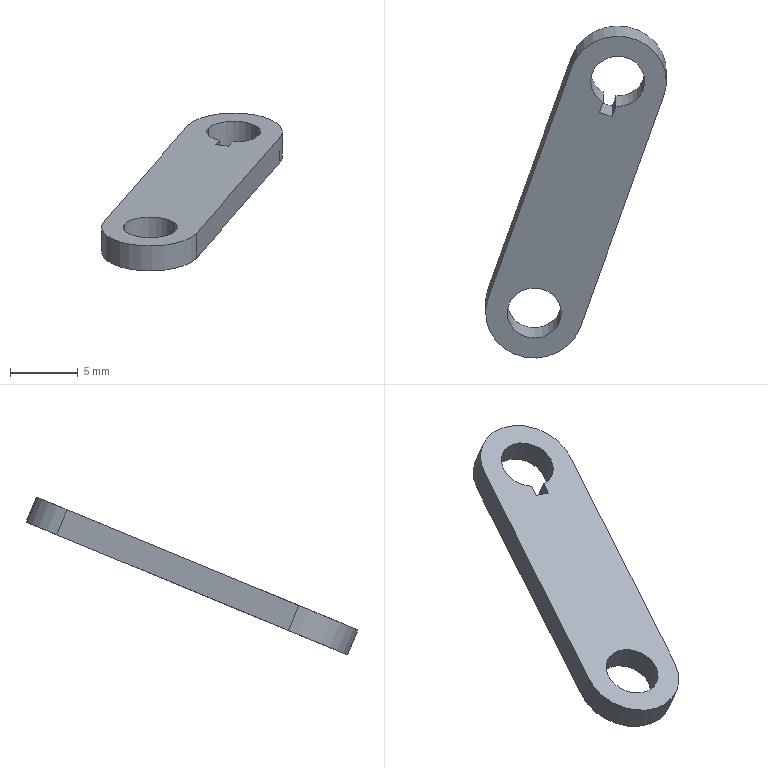Component | SolidWorks | MirrorShort Arm-2 | 1 solid | 14 faces | box 13.38 x 24.55 x 11.68 mm | volume 311 mm3 | cylinder 7 | plane 7 | commonest cylinder face diameters 4 x5 7.2 x2
STEP:
#1=CARTESIAN_POINT('',(12.305,-1.564,2.111));
#2=VERTEX_POINT('',#1);
#3=CARTESIAN_POINT('',(12.454,-1.61,2.092));
#4=VERTEX_POINT('',#3);
#5=CARTESIAN_POINT('',(12.38,-1.587,2.101));
#6=DIRECTION('',(-0.,-0.3818,0.9242));
#7=DIRECTION('',(-0.9487,0.2921,0.1207));
#8=AXIS2_PLACEMENT_3D('',#5,#6,#7);
#9=CIRCLE('',#8,0.07874);
#10=EDGE_CURVE('',#2,#4,#9,.T.);
#11=ORIENTED_EDGE('',*,*,#10,.F.);
#12=CARTESIAN_POINT('',(12.305,-1.594,2.183));
#13=VERTEX_POINT('',#12);
#14=CARTESIAN_POINT('',(12.305,-1.564,2.111));
#15=DIRECTION('',(-0.,-0.3818,0.9242));
#16=VECTOR('',#15,39.37);
#17=LINE('',#14,#16);
#18=EDGE_CURVE('',#2,#13,#17,.T.);
#19=ORIENTED_EDGE('',*,*,#18,.T.);
#20=CARTESIAN_POINT('',(12.454,-1.64,2.164));
#21=VERTEX_POINT('',#20);
#22=CARTESIAN_POINT('',(12.38,-1.617,2.174));
#23=DIRECTION('',(-0.,-0.3818,0.9242));
#24=DIRECTION('',(-0.9487,0.2921,0.1207));
#25=AXIS2_PLACEMENT_3D('',#22,#23,#24);
#26=CIRCLE('',#25,0.07874);
#27=EDGE_CURVE('',#13,#21,#26,.T.);
#28=ORIENTED_EDGE('',*,*,#27,.T.);
#29=CARTESIAN_POINT('',(12.454,-1.61,2.092));
#30=DIRECTION('',(-0.,-0.3818,0.9242));
#31=VECTOR('',#30,39.37);
#32=LINE('',#29,#31);
#33=EDGE_CURVE('',#4,#21,#32,.T.);
#34=ORIENTED_EDGE('',*,*,#33,.F.);
#35=EDGE_LOOP('',(#11,#19,#28,#34));
#36=FACE_OUTER_BOUND('',#35,.T.);
#37=CARTESIAN_POINT('',(12.38,-1.587,2.101));
#38=DIRECTION('',(-0.,-0.3818,0.9242));
#39=DIRECTION('',(0.9487,-0.2921,-0.1207));
#40=AXIS2_PLACEMENT_3D('',#37,#38,#39);
#41=CYLINDRICAL_SURFACE('',#40,0.07874);
#42=ADVANCED_FACE('',(#36),#41,.F.);
#43=CARTESIAN_POINT('',(12.548,-0.8897,2.389));
#44=VERTEX_POINT('',#43);
#45=CARTESIAN_POINT('',(12.58,-0.9738,2.354));
#46=VERTEX_POINT('',#45);
#47=CARTESIAN_POINT('',(12.623,-0.9127,2.38));
#48=DIRECTION('',(-0.,-0.3818,0.9242));
#49=DIRECTION('',(-0.9487,0.2921,0.1207));
#50=AXIS2_PLACEMENT_3D('',#47,#48,#49);
#51=CIRCLE('',#50,0.07874);
#52=EDGE_CURVE('',#44,#46,#51,.T.);
#53=ORIENTED_EDGE('',*,*,#52,.F.);
#54=CARTESIAN_POINT('',(12.548,-0.9197,2.462));
#55=VERTEX_POINT('',#54);
#56=CARTESIAN_POINT('',(12.548,-0.8897,2.389));
#57=DIRECTION('',(-0.,-0.3818,0.9242));
#58=VECTOR('',#57,39.37);
#59=LINE('',#56,#58);
#60=EDGE_CURVE('',#44,#55,#59,.T.);
#61=ORIENTED_EDGE('',*,*,#60,.T.);
#62=CARTESIAN_POINT('',(12.58,-1.004,2.427));
#63=VERTEX_POINT('',#62);
#64=CARTESIAN_POINT('',(12.623,-0.9427,2.452));
#65=DIRECTION('',(-0.,-0.3818,0.9242));
#66=DIRECTION('',(-0.9487,0.2921,0.1207));
#67=AXIS2_PLACEMENT_3D('',#64,#65,#66);
#68=CIRCLE('',#67,0.07874);
#69=EDGE_CURVE('',#55,#63,#68,.T.);
#70=ORIENTED_EDGE('',*,*,#69,.T.);
#71=CARTESIAN_POINT('',(12.58,-0.9738,2.354));
#72=DIRECTION('',(0.,0.3818,-0.9242));
#73=VECTOR('',#72,39.37);
#74=LINE('',#71,#73);
#75=EDGE_CURVE('',#63,#46,#74,.T.);
#76=ORIENTED_EDGE('',*,*,#75,.T.);
#77=EDGE_LOOP('',(#53,#61,#70,#76));
#78=FACE_OUTER_BOUND('',#77,.T.);
#79=CARTESIAN_POINT('',(12.623,-0.9127,2.38));
#80=DIRECTION('',(-0.,-0.3818,0.9242));
#81=DIRECTION('',(0.9487,-0.2921,-0.1207));
#82=AXIS2_PLACEMENT_3D('',#79,#80,#81);
#83=CYLINDRICAL_SURFACE('',#82,0.07874);
#84=ADVANCED_FACE('',(#78),#83,.F.);
#85=ORIENTED_EDGE('',*,*,#60,.F.);
#86=CARTESIAN_POINT('',(12.698,-0.9357,2.37));
#87=VERTEX_POINT('',#86);
#88=CARTESIAN_POINT('',(12.623,-0.9127,2.38));
#89=DIRECTION('',(-0.,-0.3818,0.9242));
#90=DIRECTION('',(-0.9487,0.2921,0.1207));
#91=AXIS2_PLACEMENT_3D('',#88,#89,#90);
#92=CIRCLE('',#91,0.07874);
#93=EDGE_CURVE('',#87,#44,#92,.T.);
#94=ORIENTED_EDGE('',*,*,#93,.F.);
#95=CARTESIAN_POINT('',(12.698,-0.9657,2.443));
#96=VERTEX_POINT('',#95);
#97=CARTESIAN_POINT('',(12.698,-0.9357,2.37));
#98=DIRECTION('',(-0.,-0.3818,0.9242));
#99=VECTOR('',#98,39.37);
#100=LINE('',#97,#99);
#101=EDGE_CURVE('',#87,#96,#100,.T.);
#102=ORIENTED_EDGE('',*,*,#101,.T.);
#103=CARTESIAN_POINT('',(12.623,-0.9427,2.452));
#104=DIRECTION('',(-0.,-0.3818,0.9242));
#105=DIRECTION('',(-0.9487,0.2921,0.1207));
#106=AXIS2_PLACEMENT_3D('',#103,#104,#105);
#107=CIRCLE('',#106,0.07874);
#108=EDGE_CURVE('',#96,#55,#107,.T.);
#109=ORIENTED_EDGE('',*,*,#108,.T.);
#110=EDGE_LOOP('',(#85,#94,#102,#109));
#111=FACE_OUTER_BOUND('',#110,.T.);
#112=CARTESIAN_POINT('',(12.623,-0.9127,2.38));
#113=DIRECTION('',(-0.,-0.3818,0.9242));
#114=DIRECTION('',(0.9487,-0.2921,-0.1207));
#115=AXIS2_PLACEMENT_3D('',#112,#113,#114);
#116=CYLINDRICAL_SURFACE('',#115,0.07874);
#117=ADVANCED_FACE('',(#111),#116,.F.);
#118=CARTESIAN_POINT('',(12.607,-1.015,2.337));
#119=VERTEX_POINT('',#118);
#120=CARTESIAN_POINT('',(12.617,-0.9853,2.35));
#121=VERTEX_POINT('',#120);
#122=CARTESIAN_POINT('',(12.642,-0.9184,2.377));
#123=DIRECTION('',(0.3161,0.8768,0.3623));
#124=VECTOR('',#123,39.37);
#125=LINE('',#122,#124);
#126=EDGE_CURVE('',#119,#121,#125,.T.);
#127=ORIENTED_EDGE('',*,*,#126,.T.);
#128=CARTESIAN_POINT('',(12.623,-0.9127,2.38));
#129=DIRECTION('',(-0.,-0.3818,0.9242));
#130=DIRECTION('',(-0.9487,0.2921,0.1207));
#131=AXIS2_PLACEMENT_3D('',#128,#129,#130);
#132=CIRCLE('',#131,0.07874);
#133=EDGE_CURVE('',#121,#87,#132,.T.);
#134=ORIENTED_EDGE('',*,*,#133,.T.);
#135=ORIENTED_EDGE('',*,*,#93,.T.);
#136=ORIENTED_EDGE('',*,*,#52,.T.);
#137=CARTESIAN_POINT('',(12.569,-1.004,2.342));
#138=VERTEX_POINT('',#137);
#139=CARTESIAN_POINT('',(12.604,-0.9069,2.382));
#140=DIRECTION('',(-0.3161,-0.8768,-0.3623));
#141=VECTOR('',#140,39.37);
#142=LINE('',#139,#141);
#143=EDGE_CURVE('',#46,#138,#142,.T.);
#144=ORIENTED_EDGE('',*,*,#143,.T.);
#145=CARTESIAN_POINT('',(12.588,-1.009,2.34));
#146=DIRECTION('',(0.9487,-0.2921,-0.1207));
#147=VECTOR('',#146,39.37);
#148=LINE('',#145,#147);
#149=EDGE_CURVE('',#138,#119,#148,.T.);
#150=ORIENTED_EDGE('',*,*,#149,.T.);
#151=EDGE_LOOP('',(#127,#134,#135,#136,#144,#150));
#152=FACE_BOUND('',#151,.T.);
#153=CARTESIAN_POINT('',(12.757,-0.9541,2.363));
#154=VERTEX_POINT('',#153);
#155=CARTESIAN_POINT('',(12.488,-0.8713,2.397));
#156=VERTEX_POINT('',#155);
#157=CARTESIAN_POINT('',(12.623,-0.9127,2.38));
#158=DIRECTION('',(-0.,-0.3818,0.9242));
#159=DIRECTION('',(-0.9487,0.2921,0.1207));
#160=AXIS2_PLACEMENT_3D('',#157,#158,#159);
#161=CIRCLE('',#160,0.1417);
#162=EDGE_CURVE('',#154,#156,#161,.T.);
#163=ORIENTED_EDGE('',*,*,#162,.F.);
#164=CARTESIAN_POINT('',(12.514,-1.629,2.084));
#165=VERTEX_POINT('',#164);
#166=CARTESIAN_POINT('',(12.757,-0.9541,2.363));
#167=DIRECTION('',(0.3161,0.8768,0.3623));
#168=VECTOR('',#167,39.37);
#169=LINE('',#166,#168);
#170=EDGE_CURVE('',#165,#154,#169,.T.);
#171=ORIENTED_EDGE('',*,*,#170,.F.);
#172=CARTESIAN_POINT('',(12.245,-1.546,2.118));
#173=VERTEX_POINT('',#172);
#174=CARTESIAN_POINT('',(12.38,-1.587,2.101));
#175=DIRECTION('',(-0.,-0.3818,0.9242));
#176=DIRECTION('',(-0.9487,0.2921,0.1207));
#177=AXIS2_PLACEMENT_3D('',#174,#175,#176);
#178=CIRCLE('',#177,0.1417);
#179=EDGE_CURVE('',#173,#165,#178,.T.);
#180=ORIENTED_EDGE('',*,*,#179,.F.);
#181=CARTESIAN_POINT('',(12.488,-0.8713,2.397));
#182=DIRECTION('',(-0.3161,-0.8768,-0.3623));
#183=VECTOR('',#182,39.37);
#184=LINE('',#181,#183);
#185=EDGE_CURVE('',#156,#173,#184,.T.);
#186=ORIENTED_EDGE('',*,*,#185,.F.);
#187=EDGE_LOOP('',(#163,#171,#180,#186));
#188=FACE_OUTER_BOUND('',#187,.T.);
#189=CARTESIAN_POINT('',(12.38,-1.587,2.101));
#190=DIRECTION('',(-0.,-0.3818,0.9242));
#191=DIRECTION('',(-0.9487,0.2921,0.1207));
#192=AXIS2_PLACEMENT_3D('',#189,#190,#191);
#193=CIRCLE('',#192,0.07874);
#194=EDGE_CURVE('',#4,#2,#193,.T.);
#195=ORIENTED_EDGE('',*,*,#194,.T.);
#196=ORIENTED_EDGE('',*,*,#10,.T.);
#197=EDGE_LOOP('',(#195,#196));
#198=FACE_BOUND('',#197,.T.);
#199=CARTESIAN_POINT('',(12.623,-0.9127,2.38));
#200=DIRECTION('',(0.,0.3818,-0.9242));
#201=DIRECTION('',(-0.9487,0.2921,0.1207));
#202=AXIS2_PLACEMENT_3D('',#199,#200,#201);
#203=PLANE('',#202);
#204=ADVANCED_FACE('',(#152,#188,#198),#203,.T.);
#205=CARTESIAN_POINT('',(12.757,-0.9841,2.435));
#206=VERTEX_POINT('',#205);
#207=CARTESIAN_POINT('',(12.488,-0.9013,2.47));
#208=VERTEX_POINT('',#207);
#209=CARTESIAN_POINT('',(12.623,-0.9427,2.452));
#210=DIRECTION('',(-0.,-0.3818,0.9242));
#211=DIRECTION('',(-0.9487,0.2921,0.1207));
#212=AXIS2_PLACEMENT_3D('',#209,#210,#211);
#213=CIRCLE('',#212,0.1417);
#214=EDGE_CURVE('',#206,#208,#213,.T.);
#215=ORIENTED_EDGE('',*,*,#214,.T.);
#216=CARTESIAN_POINT('',(12.245,-1.576,2.191));
#217=VERTEX_POINT('',#216);
#218=CARTESIAN_POINT('',(12.488,-0.9013,2.47));
#219=DIRECTION('',(-0.3161,-0.8768,-0.3623));
#220=VECTOR('',#219,39.37);
#221=LINE('',#218,#220);
#222=EDGE_CURVE('',#208,#217,#221,.T.);
#223=ORIENTED_EDGE('',*,*,#222,.T.);
#224=CARTESIAN_POINT('',(12.514,-1.659,2.157));
#225=VERTEX_POINT('',#224);
#226=CARTESIAN_POINT('',(12.38,-1.617,2.174));
#227=DIRECTION('',(-0.,-0.3818,0.9242));
#228=DIRECTION('',(-0.9487,0.2921,0.1207));
#229=AXIS2_PLACEMENT_3D('',#226,#227,#228);
#230=CIRCLE('',#229,0.1417);
#231=EDGE_CURVE('',#217,#225,#230,.T.);
#232=ORIENTED_EDGE('',*,*,#231,.T.);
#233=CARTESIAN_POINT('',(12.757,-0.9841,2.435));
#234=DIRECTION('',(0.3161,0.8768,0.3623));
#235=VECTOR('',#234,39.37);
#236=LINE('',#233,#235);
#237=EDGE_CURVE('',#225,#206,#236,.T.);
#238=ORIENTED_EDGE('',*,*,#237,.T.);
#239=EDGE_LOOP('',(#215,#223,#232,#238));
#240=FACE_OUTER_BOUND('',#239,.T.);
#241=CARTESIAN_POINT('',(12.569,-1.034,2.415));
#242=VERTEX_POINT('',#241);
#243=CARTESIAN_POINT('',(12.607,-1.045,2.41));
#244=VERTEX_POINT('',#243);
#245=CARTESIAN_POINT('',(12.607,-1.045,2.41));
#246=DIRECTION('',(0.9487,-0.2921,-0.1207));
#247=VECTOR('',#246,39.37);
#248=LINE('',#245,#247);
#249=EDGE_CURVE('',#242,#244,#248,.T.);
#250=ORIENTED_EDGE('',*,*,#249,.F.);
#251=CARTESIAN_POINT('',(12.604,-0.937,2.455));
#252=DIRECTION('',(-0.3161,-0.8768,-0.3623));
#253=VECTOR('',#252,39.37);
#254=LINE('',#251,#253);
#255=EDGE_CURVE('',#63,#242,#254,.T.);
#256=ORIENTED_EDGE('',*,*,#255,.F.);
#257=ORIENTED_EDGE('',*,*,#69,.F.);
#258=ORIENTED_EDGE('',*,*,#108,.F.);
#259=CARTESIAN_POINT('',(12.617,-1.015,2.422));
#260=VERTEX_POINT('',#259);
#261=CARTESIAN_POINT('',(12.623,-0.9427,2.452));
#262=DIRECTION('',(-0.,-0.3818,0.9242));
#263=DIRECTION('',(-0.9487,0.2921,0.1207));
#264=AXIS2_PLACEMENT_3D('',#261,#262,#263);
#265=CIRCLE('',#264,0.07874);
#266=EDGE_CURVE('',#260,#96,#265,.T.);
#267=ORIENTED_EDGE('',*,*,#266,.F.);
#268=CARTESIAN_POINT('',(12.642,-0.9485,2.45));
#269=DIRECTION('',(0.3161,0.8768,0.3623));
#270=VECTOR('',#269,39.37);
#271=LINE('',#268,#270);
#272=EDGE_CURVE('',#244,#260,#271,.T.);
#273=ORIENTED_EDGE('',*,*,#272,.F.);
#274=EDGE_LOOP('',(#250,#256,#257,#258,#267,#273));
#275=FACE_BOUND('',#274,.T.);
#276=CARTESIAN_POINT('',(12.38,-1.617,2.174));
#277=DIRECTION('',(-0.,-0.3818,0.9242));
#278=DIRECTION('',(-0.9487,0.2921,0.1207));
#279=AXIS2_PLACEMENT_3D('',#276,#277,#278);
#280=CIRCLE('',#279,0.07874);
#281=EDGE_CURVE('',#21,#13,#280,.T.);
#282=ORIENTED_EDGE('',*,*,#281,.F.);
#283=ORIENTED_EDGE('',*,*,#27,.F.);
#284=EDGE_LOOP('',(#282,#283));
#285=FACE_BOUND('',#284,.T.);
#286=CARTESIAN_POINT('',(12.623,-0.9427,2.452));
#287=DIRECTION('',(0.,0.3818,-0.9242));
#288=DIRECTION('',(-0.9487,0.2921,0.1207));
#289=AXIS2_PLACEMENT_3D('',#286,#287,#288);
#290=PLANE('',#289);
#291=ADVANCED_FACE('',(#240,#275,#285),#290,.F.);
#292=ORIENTED_EDGE('',*,*,#214,.F.);
#293=CARTESIAN_POINT('',(12.757,-0.9541,2.363));
#294=DIRECTION('',(-0.,-0.3818,0.9242));
#295=VECTOR('',#294,39.37);
#296=LINE('',#293,#295);
#297=EDGE_CURVE('',#154,#206,#296,.T.);
#298=ORIENTED_EDGE('',*,*,#297,.F.);
#299=ORIENTED_EDGE('',*,*,#162,.T.);
#300=CARTESIAN_POINT('',(12.488,-0.8713,2.397));
#301=DIRECTION('',(-0.,-0.3818,0.9242));
#302=VECTOR('',#301,39.37);
#303=LINE('',#300,#302);
#304=EDGE_CURVE('',#156,#208,#303,.T.);
#305=ORIENTED_EDGE('',*,*,#304,.T.);
#306=EDGE_LOOP('',(#292,#298,#299,#305));
#307=FACE_OUTER_BOUND('',#306,.T.);
#308=CARTESIAN_POINT('',(12.623,-0.9127,2.38));
#309=DIRECTION('',(-0.,-0.3818,0.9242));
#310=DIRECTION('',(0.9487,-0.2921,-0.1207));
#311=AXIS2_PLACEMENT_3D('',#308,#309,#310);
#312=CYLINDRICAL_SURFACE('',#311,0.1417);
#313=ADVANCED_FACE('',(#307),#312,.T.);
#314=ORIENTED_EDGE('',*,*,#222,.F.);
#315=ORIENTED_EDGE('',*,*,#304,.F.);
#316=ORIENTED_EDGE('',*,*,#185,.T.);
#317=CARTESIAN_POINT('',(12.245,-1.546,2.118));
#318=DIRECTION('',(-0.,-0.3818,0.9242));
#319=VECTOR('',#318,39.37);
#320=LINE('',#317,#319);
#321=EDGE_CURVE('',#173,#217,#320,.T.);
#322=ORIENTED_EDGE('',*,*,#321,.T.);
#323=EDGE_LOOP('',(#314,#315,#316,#322));
#324=FACE_OUTER_BOUND('',#323,.T.);
#325=CARTESIAN_POINT('',(12.488,-0.8713,2.397));
#326=DIRECTION('',(0.9487,-0.2921,-0.1207));
#327=DIRECTION('',(0.3161,0.8768,0.3623));
#328=AXIS2_PLACEMENT_3D('',#325,#326,#327);
#329=PLANE('',#328);
#330=ADVANCED_FACE('',(#324),#329,.F.);
#331=ORIENTED_EDGE('',*,*,#231,.F.);
#332=ORIENTED_EDGE('',*,*,#321,.F.);
#333=ORIENTED_EDGE('',*,*,#179,.T.);
#334=CARTESIAN_POINT('',(12.514,-1.629,2.084));
#335=DIRECTION('',(-0.,-0.3818,0.9242));
#336=VECTOR('',#335,39.37);
#337=LINE('',#334,#336);
#338=EDGE_CURVE('',#165,#225,#337,.T.);
#339=ORIENTED_EDGE('',*,*,#338,.T.);
#340=EDGE_LOOP('',(#331,#332,#333,#339));
#341=FACE_OUTER_BOUND('',#340,.T.);
#342=CARTESIAN_POINT('',(12.38,-1.587,2.101));
#343=DIRECTION('',(-0.,-0.3818,0.9242));
#344=DIRECTION('',(0.9487,-0.2921,-0.1207));
#345=AXIS2_PLACEMENT_3D('',#342,#343,#344);
#346=CYLINDRICAL_SURFACE('',#345,0.1417);
#347=ADVANCED_FACE('',(#341),#346,.T.);
#348=ORIENTED_EDGE('',*,*,#237,.F.);
#349=ORIENTED_EDGE('',*,*,#338,.F.);
#350=ORIENTED_EDGE('',*,*,#170,.T.);
#351=ORIENTED_EDGE('',*,*,#297,.T.);
#352=EDGE_LOOP('',(#348,#349,#350,#351));
#353=FACE_OUTER_BOUND('',#352,.T.);
#354=CARTESIAN_POINT('',(12.757,-0.9541,2.363));
#355=DIRECTION('',(-0.9487,0.2921,0.1207));
#356=DIRECTION('',(-0.3161,-0.8768,-0.3623));
#357=AXIS2_PLACEMENT_3D('',#354,#355,#356);
#358=PLANE('',#357);
#359=ADVANCED_FACE('',(#353),#358,.F.);
#360=ORIENTED_EDGE('',*,*,#101,.F.);
#361=ORIENTED_EDGE('',*,*,#133,.F.);
#362=CARTESIAN_POINT('',(12.617,-0.9853,2.35));
#363=DIRECTION('',(-0.,-0.3818,0.9242));
#364=VECTOR('',#363,39.37);
#365=LINE('',#362,#364);
#366=EDGE_CURVE('',#121,#260,#365,.T.);
#367=ORIENTED_EDGE('',*,*,#366,.T.);
#368=ORIENTED_EDGE('',*,*,#266,.T.);
#369=EDGE_LOOP('',(#360,#361,#367,#368));
#370=FACE_OUTER_BOUND('',#369,.T.);
#371=CARTESIAN_POINT('',(12.623,-0.9127,2.38));
#372=DIRECTION('',(-0.,-0.3818,0.9242));
#373=DIRECTION('',(0.9487,-0.2921,-0.1207));
#374=AXIS2_PLACEMENT_3D('',#371,#372,#373);
#375=CYLINDRICAL_SURFACE('',#374,0.07874);
#376=ADVANCED_FACE('',(#370),#375,.F.);
#377=ORIENTED_EDGE('',*,*,#18,.F.);
#378=ORIENTED_EDGE('',*,*,#194,.F.);
#379=ORIENTED_EDGE('',*,*,#33,.T.);
#380=ORIENTED_EDGE('',*,*,#281,.T.);
#381=EDGE_LOOP('',(#377,#378,#379,#380));
#382=FACE_OUTER_BOUND('',#381,.T.);
#383=CARTESIAN_POINT('',(12.38,-1.587,2.101));
#384=DIRECTION('',(-0.,-0.3818,0.9242));
#385=DIRECTION('',(0.9487,-0.2921,-0.1207));
#386=AXIS2_PLACEMENT_3D('',#383,#384,#385);
#387=CYLINDRICAL_SURFACE('',#386,0.07874);
#388=ADVANCED_FACE('',(#382),#387,.F.);
#389=ORIENTED_EDGE('',*,*,#126,.F.);
#390=CARTESIAN_POINT('',(12.607,-1.045,2.41));
#391=DIRECTION('',(0.,0.3818,-0.9242));
#392=VECTOR('',#391,39.37);
#393=LINE('',#390,#392);
#394=EDGE_CURVE('',#244,#119,#393,.T.);
#395=ORIENTED_EDGE('',*,*,#394,.F.);
#396=ORIENTED_EDGE('',*,*,#272,.T.);
#397=ORIENTED_EDGE('',*,*,#366,.F.);
#398=EDGE_LOOP('',(#389,#395,#396,#397));
#399=FACE_OUTER_BOUND('',#398,.T.);
#400=CARTESIAN_POINT('',(12.642,-0.9485,2.45));
#401=DIRECTION('',(0.9487,-0.2921,-0.1207));
#402=DIRECTION('',(0.3161,0.8768,0.3623));
#403=AXIS2_PLACEMENT_3D('',#400,#401,#402);
#404=PLANE('',#403);
#405=ADVANCED_FACE('',(#399),#404,.F.);
#406=ORIENTED_EDGE('',*,*,#149,.F.);
#407=CARTESIAN_POINT('',(12.569,-1.034,2.415));
#408=DIRECTION('',(0.,0.3818,-0.9242));
#409=VECTOR('',#408,39.37);
#410=LINE('',#407,#409);
#411=EDGE_CURVE('',#242,#138,#410,.T.);
#412=ORIENTED_EDGE('',*,*,#411,.F.);
#413=ORIENTED_EDGE('',*,*,#249,.T.);
#414=ORIENTED_EDGE('',*,*,#394,.T.);
#415=EDGE_LOOP('',(#406,#412,#413,#414));
#416=FACE_OUTER_BOUND('',#415,.T.);
#417=CARTESIAN_POINT('',(12.607,-1.045,2.41));
#418=DIRECTION('',(-0.3161,-0.8768,-0.3623));
#419=DIRECTION('',(0.9487,-0.2921,-0.1207));
#420=AXIS2_PLACEMENT_3D('',#417,#418,#419);
#421=PLANE('',#420);
#422=ADVANCED_FACE('',(#416),#421,.F.);
#423=ORIENTED_EDGE('',*,*,#143,.F.);
#424=ORIENTED_EDGE('',*,*,#75,.F.);
#425=ORIENTED_EDGE('',*,*,#255,.T.);
#426=ORIENTED_EDGE('',*,*,#411,.T.);
#427=EDGE_LOOP('',(#423,#424,#425,#426));
#428=FACE_OUTER_BOUND('',#427,.T.);
#429=CARTESIAN_POINT('',(12.604,-0.937,2.455));
#430=DIRECTION('',(-0.9487,0.2921,0.1207));
#431=DIRECTION('',(-0.3161,-0.8768,-0.3623));
#432=AXIS2_PLACEMENT_3D('',#429,#430,#431);
#433=PLANE('',#432);
#434=ADVANCED_FACE('',(#428),#433,.F.);
#435=CLOSED_SHELL('',(#42,#84,#117,#204,#291,#313,#330,#347,#359,#376,#388,#405,#422,#434));
#436=MANIFOLD_SOLID_BREP('',#435);
#437=CARTESIAN_POINT('',(0.,0.,0.));
#438=DIRECTION('',(0.,0.,1.));
#439=DIRECTION('',(1.,0.,0.));
#440=AXIS2_PLACEMENT_3D('',#437,#438,#439);
#441=(LENGTH_UNIT()NAMED_UNIT(*)SI_UNIT($,.METRE.));
#442=LENGTH_MEASURE_WITH_UNIT(LENGTH_MEASURE(0.0254),#441);
#443=DIMENSIONAL_EXPONENTS(1.,0.,0.,0.,0.,0.,0.);
#444=(CONVERSION_BASED_UNIT('',#442)LENGTH_UNIT()NAMED_UNIT(#443));
#445=UNCERTAINTY_MEASURE_WITH_UNIT(LENGTH_MEASURE(0.00001),#444,'','');
#446=(NAMED_UNIT(*)PLANE_ANGLE_UNIT()SI_UNIT($,.RADIAN.));
#447=(NAMED_UNIT(*)SI_UNIT($,.STERADIAN.)SOLID_ANGLE_UNIT());
#448=(GEOMETRIC_REPRESENTATION_CONTEXT(3)GLOBAL_UNCERTAINTY_ASSIGNED_CONTEXT((#445))GLOBAL_UNIT_ASSIGNED_CONTEXT((#444,#446,#447))REPRESENTATION_CONTEXT('',''));
#449=ADVANCED_BREP_SHAPE_REPRESENTATION('',(#436,#440),#448);
#450=COLOUR_RGB('',0.7922,0.8196,0.9333);
#451=FILL_AREA_STYLE_COLOUR('',#450);
#452=FILL_AREA_STYLE('',(#451));
#453=SURFACE_STYLE_FILL_AREA(#452);
#454=SURFACE_SIDE_STYLE('',(#453));
#455=SURFACE_STYLE_USAGE(.BOTH.,#454);
#456=PRESENTATION_STYLE_ASSIGNMENT((#455));
#457=STYLED_ITEM('',(#456),#436);
#458=PRESENTATION_LAYER_ASSIGNMENT('','',(#457));
#459=(LENGTH_UNIT()NAMED_UNIT(*)SI_UNIT($,.METRE.));
#460=LENGTH_MEASURE_WITH_UNIT(LENGTH_MEASURE(0.0254),#459);
#461=DIMENSIONAL_EXPONENTS(1.,0.,0.,0.,0.,0.,0.);
#462=(CONVERSION_BASED_UNIT('',#460)LENGTH_UNIT()NAMED_UNIT(#461));
#463=UNCERTAINTY_MEASURE_WITH_UNIT(LENGTH_MEASURE(0.00001),#462,'','');
#464=(NAMED_UNIT(*)PLANE_ANGLE_UNIT()SI_UNIT($,.RADIAN.));
#465=(NAMED_UNIT(*)SI_UNIT($,.STERADIAN.)SOLID_ANGLE_UNIT());
#466=(GEOMETRIC_REPRESENTATION_CONTEXT(3)GLOBAL_UNCERTAINTY_ASSIGNED_CONTEXT((#463))GLOBAL_UNIT_ASSIGNED_CONTEXT((#462,#464,#465))REPRESENTATION_CONTEXT('',''));
#467=MECHANICAL_DESIGN_GEOMETRIC_PRESENTATION_REPRESENTATION('',(#457),#466);